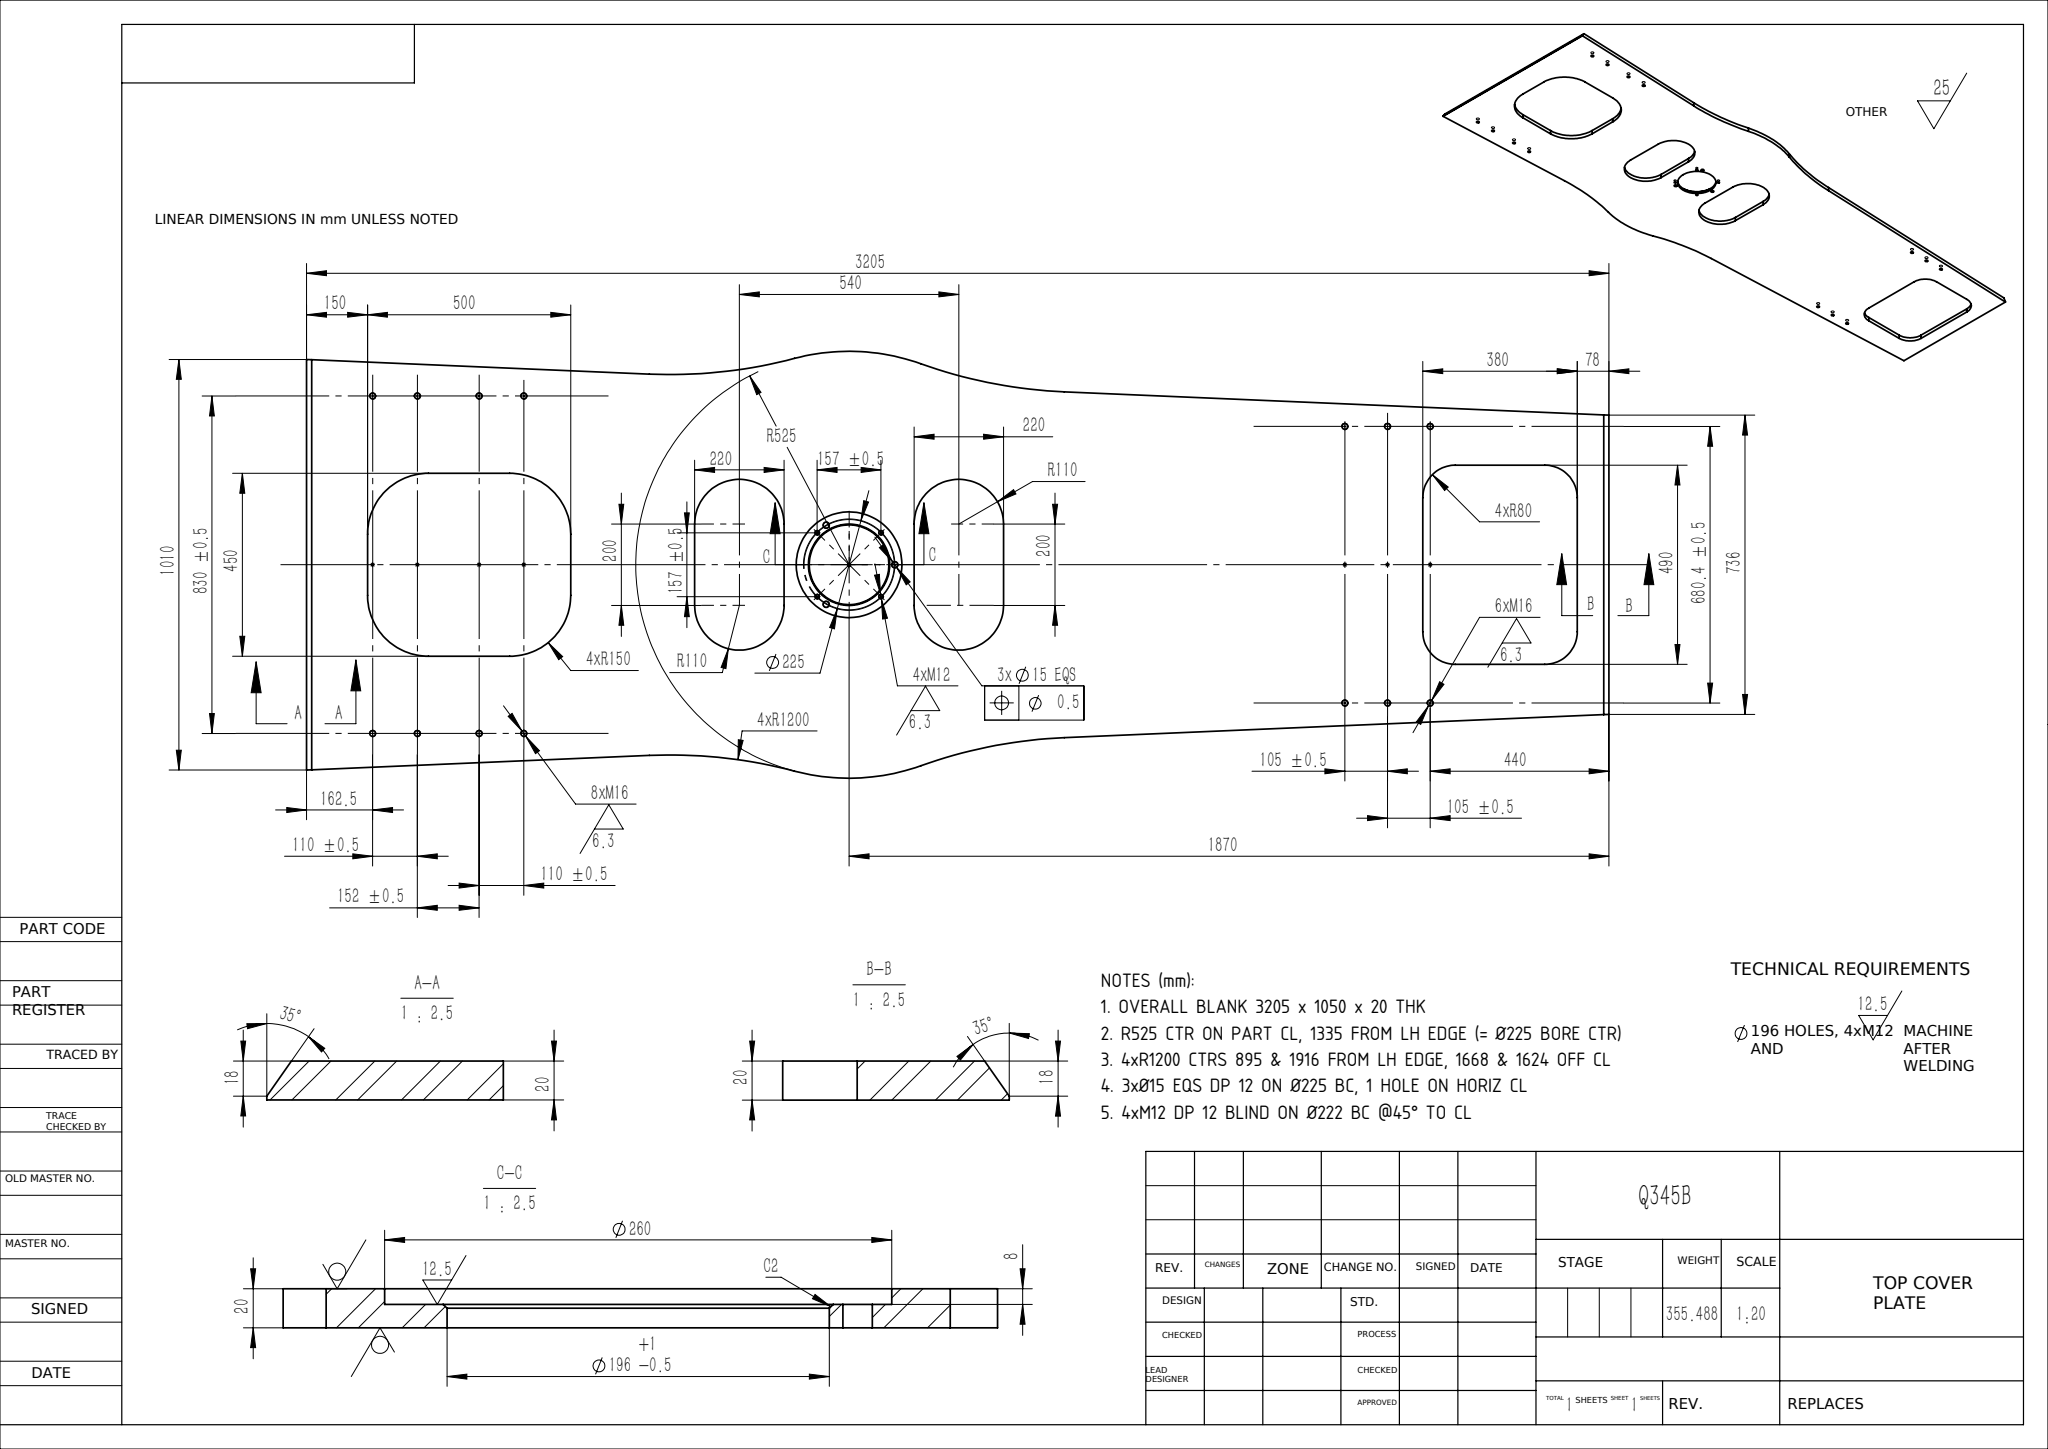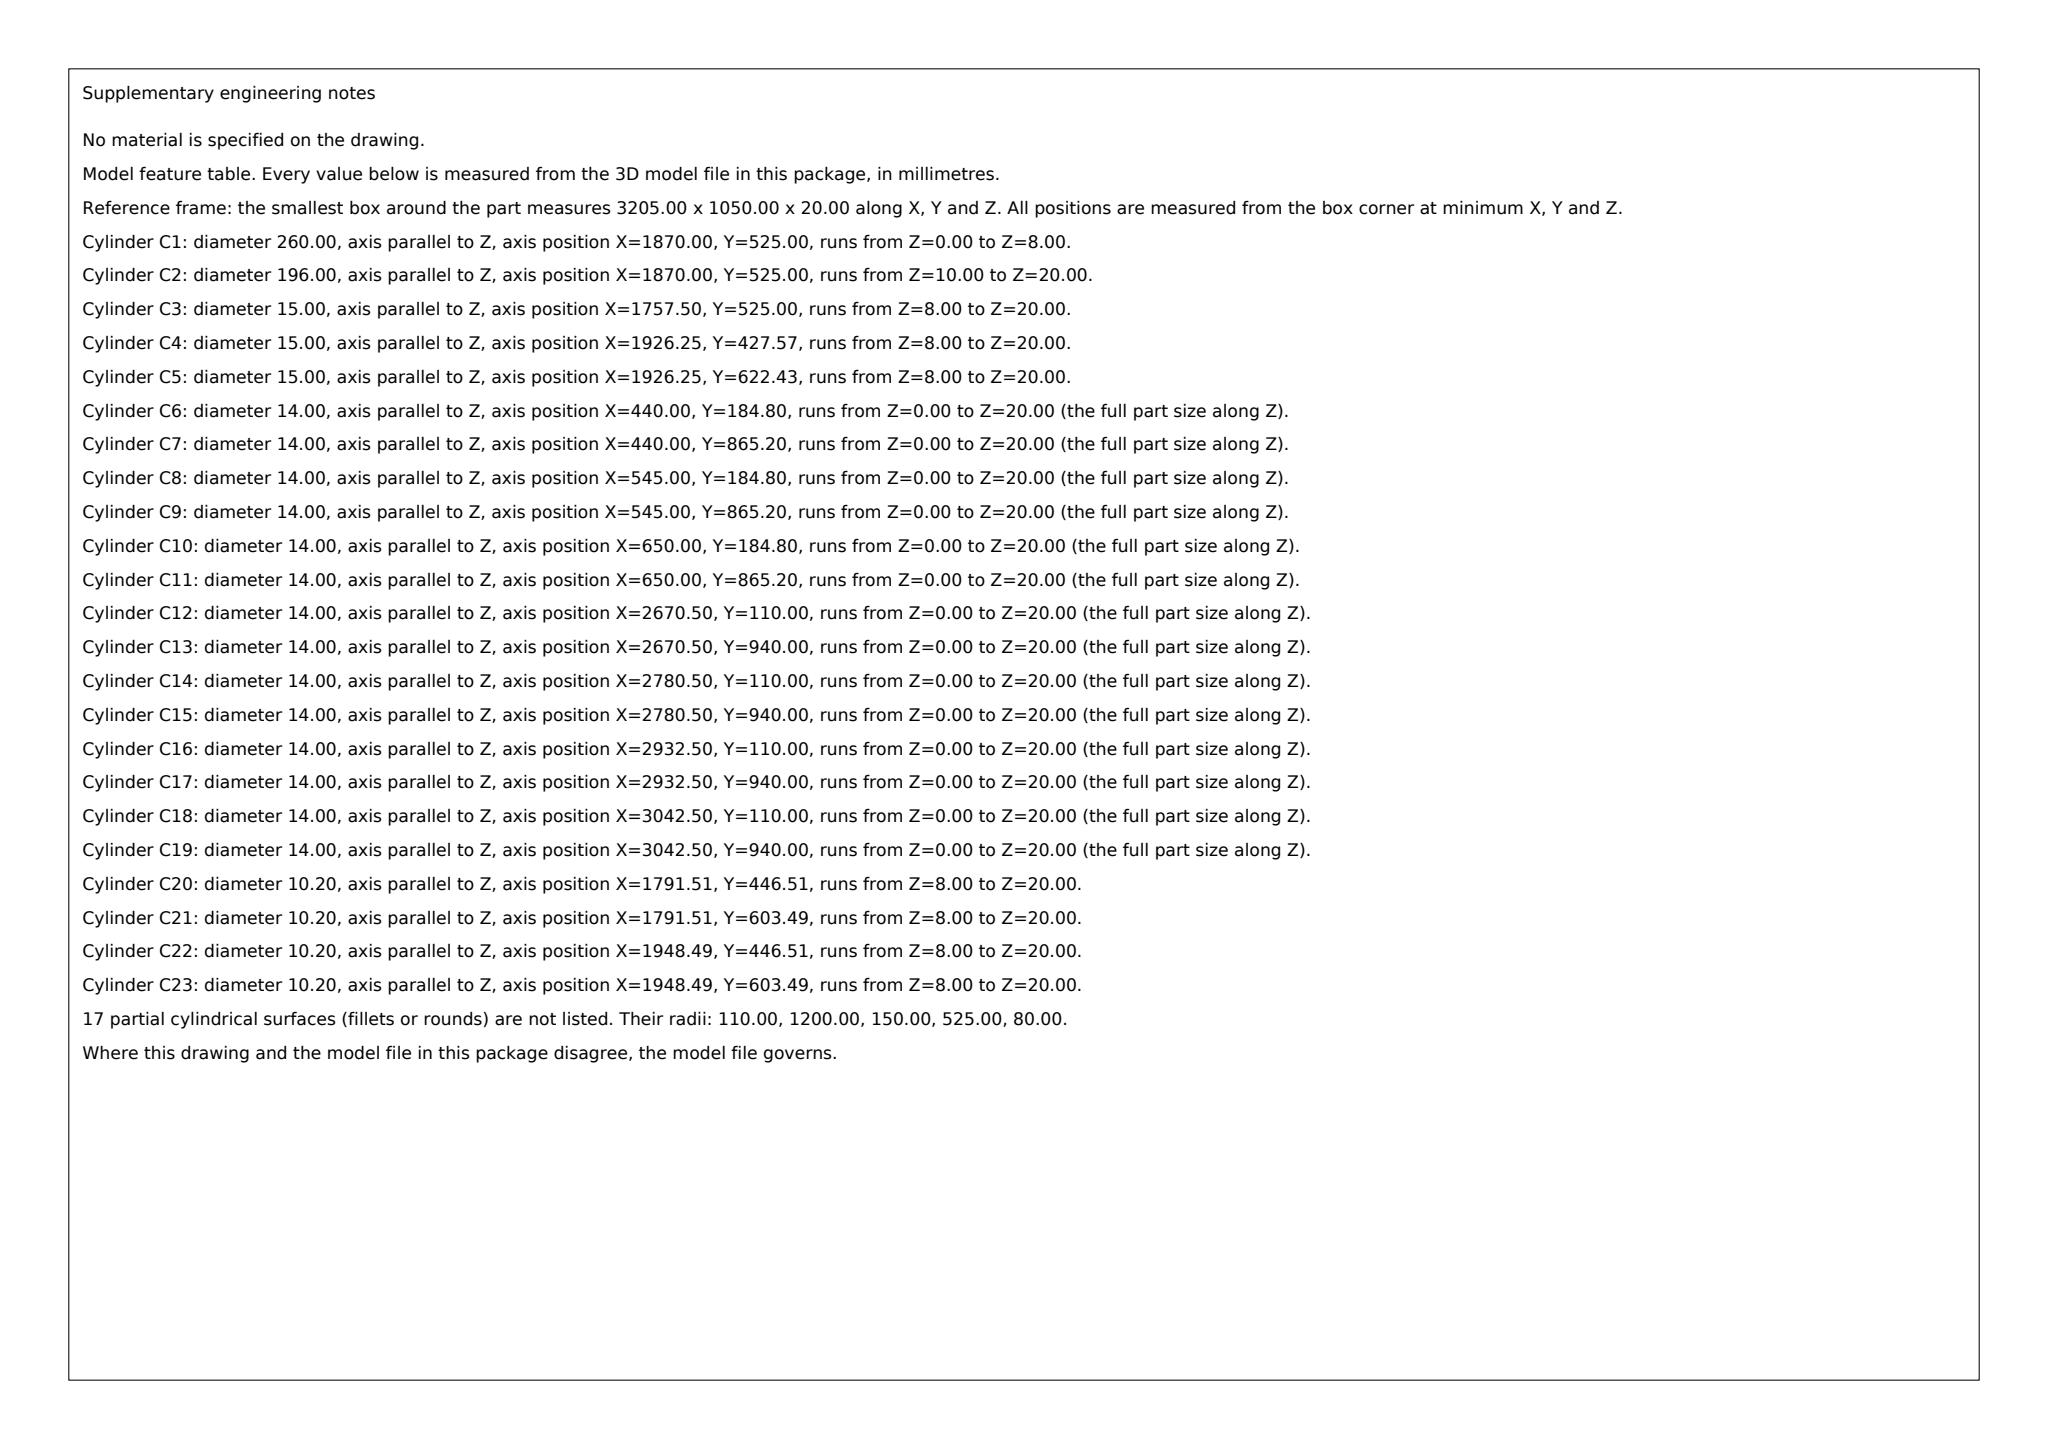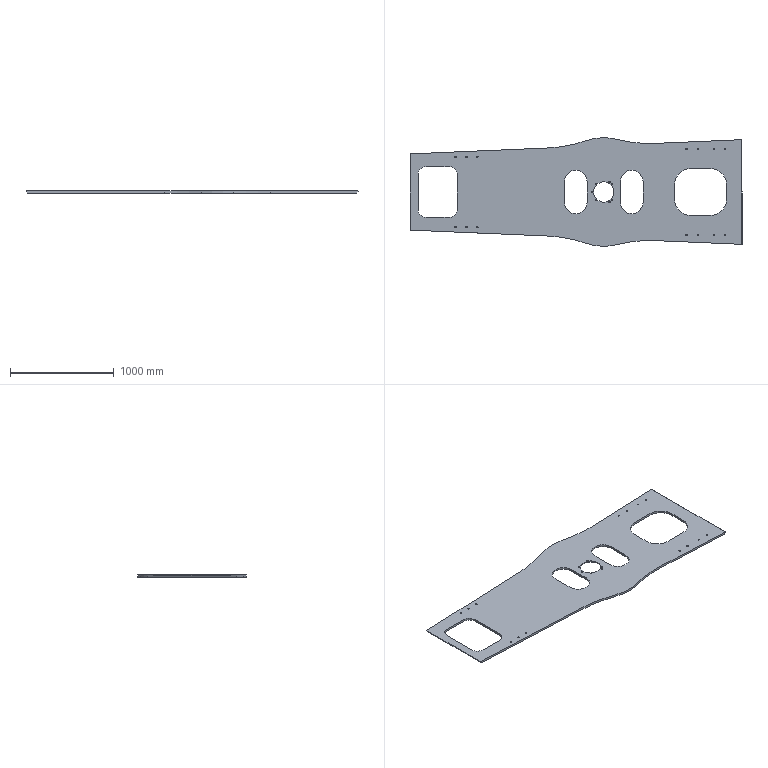Part | SolidWorks | mm | 1 solid | 89 faces | box 3205 x 1050 x 20 mm | volume 45285105 mm3 | cylinder 64 | plane 23 | cone 2 | commonest cylinder face diameters 14 x28 10.2 x8 15 x6 2400 x4 220 x4 160 x4 300 x4 260 x2
Drawing notes:
OVERALL BLANK 3205 x 1050 x 20 THK | from the solid: bbox_xyz 3205 x 1050 x 20
R525 CTR ON PART CL, 1335 FROM LH EDGE (= Ø225 BORE CTR) | from the solid: cyl dia 1050 (R525) axis z at x=1870, y=525; 3205-1870=1335 from LH edge; CL y=525
4xR1200 CTRS 895 & 1916 FROM LH EDGE, 1668 & 1624 OFF CL | from the solid: dia 2400 cyls at (2310.33,-1142.85),(2310.33,2192.85),(1288.95,-1099.19),(1288.95,2149.19)
3xØ15 EQS DP 12 ON Ø225 BC, 1 HOLE ON HORIZ CL | from the solid: Ø15 z-cyls L=12 at (1757.5,525),(1926.25,427.57),(1926.25,622.43), R112.5 about (1870,525)
4xM12 DP 12 BLIND ON Ø222 BC @45° TO CL | from the solid: Ø10.2 z-cyls L=12 at (1791.51/1948.49, 446.51/603.49) = R111 about bore ctr; plate 20 thk
build123d program:
from build123d import *

# Parameters (mm, degrees)
SKETCH1_R               = 98
BOSS_EXTRUDE1_DEPTH     = 20
SKETCH2_R               = 130
CUT_EXTRUDE2_DEPTH      = 8
M12_TAPPED_HOLE1_D      = 10.2
M16_TAPPED_HOLE2_D      = 14
M16_TAPPED_HOLE3_D      = 14
CHAMFER1_SIZE           = 2
CUT_EXTRUDE5_DEPTH      = 2015.895
CUT_EXTRUDE5_DEPTH_BACK = 2015.895
SKETCH3_R               = 7.5
CUT_EXTRUDE6_DEPTH      = 1943.336


with BuildPart() as part:
    # Sketch1 → Boss-Extrude1 (new body)
    with BuildSketch(Plane.XY):
        with BuildLine():
            Line((1335, -505), (1335, 505))
            Line((1335, 505), (491.58, 468.947))
            ThreePointArc((491.58, 468.947), (311.341, 474.806), (134.014, 507.607))
            ThreePointArc((134.014, 507.607), (-22.421, 524.521), (-176.842, 494.32))
            ThreePointArc((-176.842, 494.32), (-350.723, 446.505), (-529.805, 425.288))
            Line((-529.805, 425.288), (-1870, 368))
            Line((-1870, 368), (-1870, -368))
            Line((-1870, -368), (-529.805, -425.288))
            ThreePointArc((-529.805, -425.288), (-350.723, -446.505), (-176.842, -494.32))
            ThreePointArc((-176.842, -494.32), (-22.421, -524.521), (134.014, -507.607))
            ThreePointArc((134.014, -507.607), (311.341, -474.806), (491.58, -468.947))
            Line((491.58, -468.947), (1335, -505))
        make_face()
        Circle(SKETCH1_R, mode=Mode.SUBTRACT)
        with BuildLine():
            Line((1185, -75), (1185, 75))
            ThreePointArc((1185, 75), (1141.066, 181.066), (1035, 225))
            Line((1035, 225), (835, 225))
            ThreePointArc((835, 225), (728.934, 181.066), (685, 75))
            Line((685, 75), (685, -75))
            ThreePointArc((685, -75), (728.934, -181.066), (835, -225))
            Line((835, -225), (1035, -225))
            ThreePointArc((1035, -225), (1141.066, -181.066), (1185, -75))
        make_face(mode=Mode.SUBTRACT)
        with BuildLine():
            Line((-1412, -165), (-1412, 165))
            ThreePointArc((-1412, 165), (-1435.431, 221.569), (-1492, 245))
            Line((-1492, 245), (-1712, 245))
            ThreePointArc((-1712, 245), (-1768.569, 221.569), (-1792, 165))
            Line((-1792, 165), (-1792, -165))
            ThreePointArc((-1792, -165), (-1768.569, -221.569), (-1712, -245))
            Line((-1712, -245), (-1492, -245))
            ThreePointArc((-1492, -245), (-1435.431, -221.569), (-1412, -165))
        make_face(mode=Mode.SUBTRACT)
        with BuildLine():
            Line((160, 100), (160, -100))
            ThreePointArc((160, -100), (270, -210), (380, -100))
            Line((380, -100), (380, 100))
            ThreePointArc((380, 100), (270, 210), (160, 100))
        make_face(mode=Mode.SUBTRACT)
        with BuildLine():
            Line((-160, 100), (-160, -100))
            ThreePointArc((-160, -100), (-270, -210), (-380, -100))
            Line((-380, -100), (-380, 100))
            ThreePointArc((-380, 100), (-270, 210), (-160, 100))
        make_face(mode=Mode.SUBTRACT)
    extrude(amount=BOSS_EXTRUDE1_DEPTH)

    # Sketch2 → Cut-Extrude2 (cut)
    with BuildSketch(Plane.XY):
        Circle(SKETCH2_R)
    extrude(amount=CUT_EXTRUDE2_DEPTH, mode=Mode.SUBTRACT)

    # M12 Tapped Hole1 (through all)
    with Locations(Plane(origin=(78.489, 78.489, 8), x_dir=(-1, 0, 0), z_dir=(0, 0, -1))):
        with Locations((0, 0), (156.978, 0), (156.978, -156.978), (0, -156.978)):
            Hole(M12_TAPPED_HOLE1_D / 2)

    # M16 Tapped Hole2 (through all)
    with Locations(Plane(origin=(0, 0, 0), x_dir=(-1, 0, 0), z_dir=(0, 0, -1))):
        with Locations((-1172.5, 415)):
            Hole(M16_TAPPED_HOLE2_D / 2)

    # M16 Tapped Hole3 (through all)
    with Locations(Plane(origin=(0, 0, 0), x_dir=(-1, 0, 0), z_dir=(0, 0, -1))):
        with Locations((-1062.5, 415), (-910.5, 415), (-800.5, 415), (-1172.5, -415), (-1062.5, -415), (-910.5, -415), (-800.5, -415), (1220, 340.2), (1325, 340.2), (1430, 340.2), (1220, -340.2), (1325, -340.2), (1430, -340.2)):
            Hole(M16_TAPPED_HOLE3_D / 2)

    # Chamfer1
    chamfer1_edges = [part.edges().sort_by_distance(p)[0] for p in [
        (-98, 0, 8),
    ]]
    chamfer(chamfer1_edges, length=CHAMFER1_SIZE)

    # Sketch21 → Cut-Extrude5 (cut, two sides: drawn at the far end of the back side and taken through both)
    with BuildSketch(Plane.XZ.offset(-225).offset(-CUT_EXTRUDE5_DEPTH_BACK)):
        Polygon((-1870, 18), (-1857.396, 0), (-1870, 0), align=None)
        Polygon((1335, 18), (1322.396, 0), (1335, 0), align=None)
    extrude(amount=CUT_EXTRUDE5_DEPTH + CUT_EXTRUDE5_DEPTH_BACK, mode=Mode.SUBTRACT)

    # Sketch3 → Cut-Extrude6 (cut, through all)
    with BuildSketch(Plane(origin=(0, 0, 8), x_dir=(-1, 0, 0), z_dir=(0, 0, -1))):
        with Locations((112.5, 0)):
            Circle(SKETCH3_R)
        with Locations((-56.25, -97.428)):
            Circle(SKETCH3_R)
        with Locations((-56.25, 97.428)):
            Circle(SKETCH3_R)
    extrude(amount=-CUT_EXTRUDE6_DEPTH, mode=Mode.SUBTRACT)


solid = part.part